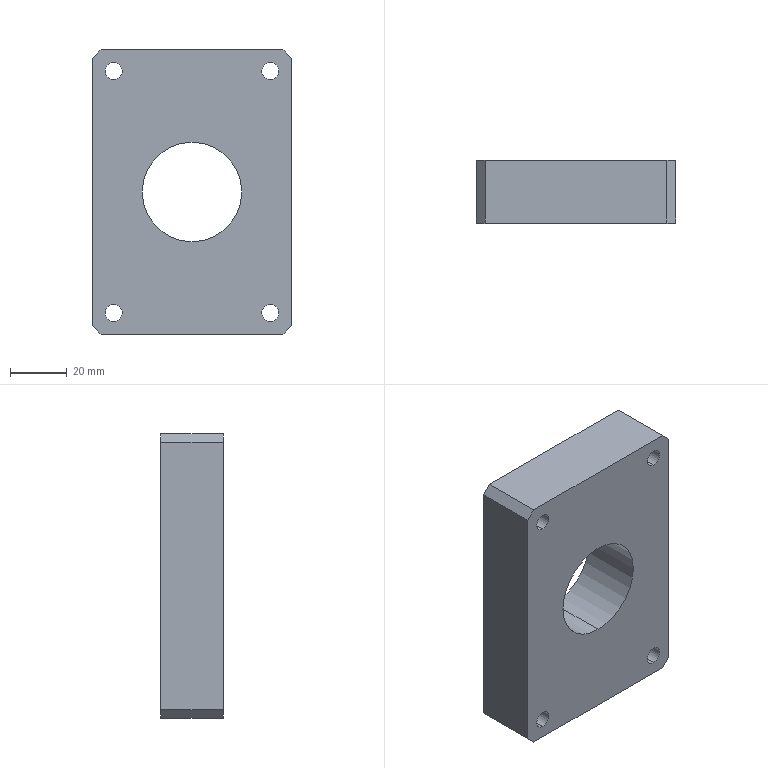Component | SolidWorks | CounterMountingPlate-1 | 1 solid | 35 faces | box 70 x 22 x 100 mm | volume 128818 mm3 | cylinder 20 | plane 15 | commonest cylinder face diameters 6 x10 9 x8 35 x2
build123d program:
from build123d import *

# Parameters (mm, degrees)
SKETCH1_W                                           = 70
SKETCH1_H                                           = 100
BOSS_EXTRUDE1_DEPTH                                 = 22
SKETCH2_R                                           = 17.5
CUT_EXTRUDE1_DEPTH                                  = 65.877
CYLINDRICAL_COUNTERSUNK_HOLE_FOR_M5_HEX_D           = 6
CYLINDRICAL_COUNTERSUNK_HOLE_FOR_M5_HEX_CBORE_D     = 9
CYLINDRICAL_COUNTERSUNK_HOLE_FOR_M5_HEX_CBORE_DEPTH = 6
CHAMFER1_SIZE                                       = 3
SKETCH8_R                                           = 3
CUT_EXTRUDE2_DEPTH                                  = 10


with BuildPart() as part:
    # Sketch1 → Boss-Extrude1 (new body)
    with BuildSketch(Plane(origin=(0, 0, 0), x_dir=(1, 0, 0), z_dir=(0, 1, 0))):
        Rectangle(SKETCH1_W, SKETCH1_H)
    extrude(amount=BOSS_EXTRUDE1_DEPTH)

    # Sketch2 → Cut-Extrude1 (cut, through all)
    with BuildSketch(Plane.XZ):
        with Locations(Location((0, 0, 0), (0, 0, 270))):
            Circle(SKETCH2_R)
    extrude(amount=-CUT_EXTRUDE1_DEPTH, mode=Mode.SUBTRACT)

    # Cylindrical Countersunk Hole for M5 Hex (through all)
    with Locations(Plane(origin=(0, 22, 0), x_dir=(1, 0, 0), z_dir=(0, 1, 0))):
        with Locations((-27.5, 42.5), (27.5, 42.5), (27.5, -42.5), (-27.5, -42.5)):
            CounterBoreHole(CYLINDRICAL_COUNTERSUNK_HOLE_FOR_M5_HEX_D / 2, CYLINDRICAL_COUNTERSUNK_HOLE_FOR_M5_HEX_CBORE_D / 2, CYLINDRICAL_COUNTERSUNK_HOLE_FOR_M5_HEX_CBORE_DEPTH)

    # Chamfer1
    chamfer1_edges = [part.edges().sort_by_distance(p)[0] for p in [
        (35, 11, 50),
        (-35, 11, 50),
        (-35, 11, -50),
        (35, 11, -50),
    ]]
    chamfer(chamfer1_edges, length=CHAMFER1_SIZE)

    # Sketch8 → Cut-Extrude2 (cut)
    with BuildSketch(Plane(origin=(0, 22, 0), x_dir=(1, 0, 0), z_dir=(0, 1, 0))):
        with Locations(Location((0, -30, 0), (0, 0, 270))):
            Circle(SKETCH8_R)
    extrude(amount=-CUT_EXTRUDE2_DEPTH, mode=Mode.SUBTRACT)


solid = part.part

# Placed as in the assembly
solid = solid.moved(Location((-29.507, 247.589, 458), (0, 0, 0)))
STEP:
#1=COLOUR_RGB('',0.7922,0.8196,0.9333);
#2=FILL_AREA_STYLE_COLOUR('',#1);
#3=FILL_AREA_STYLE('',(#2));
#4=SURFACE_STYLE_FILL_AREA(#3);
#5=SURFACE_SIDE_STYLE('',(#4));
#6=SURFACE_STYLE_USAGE(.BOTH.,#5);
#7=PRESENTATION_STYLE_ASSIGNMENT((#6));
#8=CARTESIAN_POINT('',(-1.162,10.22,19.094));
#9=VERTEX_POINT('',#8);
#10=CARTESIAN_POINT('',(-1.162,10.22,19.331));
#11=VERTEX_POINT('',#10);
#12=CARTESIAN_POINT('',(-1.162,10.22,19.213));
#13=DIRECTION('',(0.,1.,0.));
#14=DIRECTION('',(0.,0.,1.));
#15=AXIS2_PLACEMENT_3D('',#12,#13,#14);
#16=CIRCLE('',#15,0.1181);
#17=EDGE_CURVE('',#9,#11,#16,.T.);
#18=ORIENTED_EDGE('',*,*,#17,.F.);
#19=CARTESIAN_POINT('',(-1.162,10.614,19.094));
#20=VERTEX_POINT('',#19);
#21=CARTESIAN_POINT('',(-1.162,10.22,19.094));
#22=DIRECTION('',(0.,1.,0.));
#23=VECTOR('',#22,39.37);
#24=LINE('',#21,#23);
#25=EDGE_CURVE('',#9,#20,#24,.T.);
#26=ORIENTED_EDGE('',*,*,#25,.T.);
#27=CARTESIAN_POINT('',(-1.162,10.614,19.331));
#28=VERTEX_POINT('',#27);
#29=CARTESIAN_POINT('',(-1.162,10.614,19.213));
#30=DIRECTION('',(0.,1.,0.));
#31=DIRECTION('',(0.,0.,1.));
#32=AXIS2_PLACEMENT_3D('',#29,#30,#31);
#33=CIRCLE('',#32,0.1181);
#34=EDGE_CURVE('',#20,#28,#33,.T.);
#35=ORIENTED_EDGE('',*,*,#34,.T.);
#36=CARTESIAN_POINT('',(-1.162,10.22,19.331));
#37=DIRECTION('',(0.,1.,0.));
#38=VECTOR('',#37,39.37);
#39=LINE('',#36,#38);
#40=EDGE_CURVE('',#11,#28,#39,.T.);
#41=ORIENTED_EDGE('',*,*,#40,.F.);
#42=EDGE_LOOP('',(#18,#26,#35,#41));
#43=FACE_OUTER_BOUND('',#42,.T.);
#44=CARTESIAN_POINT('',(-1.162,10.22,19.213));
#45=DIRECTION('',(0.,1.,0.));
#46=DIRECTION('',(0.,0.,1.));
#47=AXIS2_PLACEMENT_3D('',#44,#45,#46);
#48=CYLINDRICAL_SURFACE('',#47,0.1181);
#49=ADVANCED_FACE('',(#43),#48,.F.);
#50=CARTESIAN_POINT('',(-2.244,10.378,16.181));
#51=VERTEX_POINT('',#50);
#52=CARTESIAN_POINT('',(-2.244,10.378,16.535));
#53=VERTEX_POINT('',#52);
#54=CARTESIAN_POINT('',(-2.244,10.378,16.358));
#55=DIRECTION('',(0.,1.,0.));
#56=DIRECTION('',(0.,0.,1.));
#57=AXIS2_PLACEMENT_3D('',#54,#55,#56);
#58=CIRCLE('',#57,0.1772);
#59=EDGE_CURVE('',#51,#53,#58,.T.);
#60=ORIENTED_EDGE('',*,*,#59,.F.);
#61=CARTESIAN_POINT('',(-2.244,10.614,16.181));
#62=VERTEX_POINT('',#61);
#63=CARTESIAN_POINT('',(-2.244,10.614,16.181));
#64=DIRECTION('',(0.,1.,0.));
#65=VECTOR('',#64,39.37);
#66=LINE('',#63,#65);
#67=EDGE_CURVE('',#51,#62,#66,.T.);
#68=ORIENTED_EDGE('',*,*,#67,.T.);
#69=CARTESIAN_POINT('',(-2.244,10.614,16.535));
#70=VERTEX_POINT('',#69);
#71=CARTESIAN_POINT('',(-2.244,10.614,16.358));
#72=DIRECTION('',(0.,1.,0.));
#73=DIRECTION('',(0.,0.,1.));
#74=AXIS2_PLACEMENT_3D('',#71,#72,#73);
#75=CIRCLE('',#74,0.1772);
#76=EDGE_CURVE('',#62,#70,#75,.T.);
#77=ORIENTED_EDGE('',*,*,#76,.T.);
#78=CARTESIAN_POINT('',(-2.244,10.614,16.535));
#79=DIRECTION('',(0.,1.,0.));
#80=VECTOR('',#79,39.37);
#81=LINE('',#78,#80);
#82=EDGE_CURVE('',#53,#70,#81,.T.);
#83=ORIENTED_EDGE('',*,*,#82,.F.);
#84=EDGE_LOOP('',(#60,#68,#77,#83));
#85=FACE_OUTER_BOUND('',#84,.T.);
#86=CARTESIAN_POINT('',(-2.244,10.614,16.358));
#87=DIRECTION('',(0.,1.,0.));
#88=DIRECTION('',(0.,0.,1.));
#89=AXIS2_PLACEMENT_3D('',#86,#87,#88);
#90=CYLINDRICAL_SURFACE('',#89,0.1772);
#91=ADVANCED_FACE('',(#85),#90,.F.);
#92=CARTESIAN_POINT('',(-2.244,9.748,16.24));
#93=VERTEX_POINT('',#92);
#94=CARTESIAN_POINT('',(-2.244,9.748,16.476));
#95=VERTEX_POINT('',#94);
#96=CARTESIAN_POINT('',(-2.244,9.748,16.358));
#97=DIRECTION('',(0.,1.,0.));
#98=DIRECTION('',(0.,0.,1.));
#99=AXIS2_PLACEMENT_3D('',#96,#97,#98);
#100=CIRCLE('',#99,0.1181);
#101=EDGE_CURVE('',#93,#95,#100,.T.);
#102=ORIENTED_EDGE('',*,*,#101,.F.);
#103=CARTESIAN_POINT('',(-2.244,10.378,16.24));
#104=VERTEX_POINT('',#103);
#105=CARTESIAN_POINT('',(-2.244,10.614,16.24));
#106=DIRECTION('',(0.,1.,0.));
#107=VECTOR('',#106,39.37);
#108=LINE('',#105,#107);
#109=EDGE_CURVE('',#93,#104,#108,.T.);
#110=ORIENTED_EDGE('',*,*,#109,.T.);
#111=CARTESIAN_POINT('',(-2.244,10.378,16.476));
#112=VERTEX_POINT('',#111);
#113=CARTESIAN_POINT('',(-2.244,10.378,16.358));
#114=DIRECTION('',(0.,1.,0.));
#115=DIRECTION('',(0.,0.,1.));
#116=AXIS2_PLACEMENT_3D('',#113,#114,#115);
#117=CIRCLE('',#116,0.1181);
#118=EDGE_CURVE('',#104,#112,#117,.T.);
#119=ORIENTED_EDGE('',*,*,#118,.T.);
#120=CARTESIAN_POINT('',(-2.244,10.614,16.476));
#121=DIRECTION('',(0.,1.,0.));
#122=VECTOR('',#121,39.37);
#123=LINE('',#120,#122);
#124=EDGE_CURVE('',#95,#112,#123,.T.);
#125=ORIENTED_EDGE('',*,*,#124,.F.);
#126=EDGE_LOOP('',(#102,#110,#119,#125));
#127=FACE_OUTER_BOUND('',#126,.T.);
#128=CARTESIAN_POINT('',(-2.244,10.614,16.358));
#129=DIRECTION('',(0.,1.,0.));
#130=DIRECTION('',(0.,0.,1.));
#131=AXIS2_PLACEMENT_3D('',#128,#129,#130);
#132=CYLINDRICAL_SURFACE('',#131,0.1181);
#133=ADVANCED_FACE('',(#127),#132,.F.);
#134=CARTESIAN_POINT('',(-0.079,10.378,16.181));
#135=VERTEX_POINT('',#134);
#136=CARTESIAN_POINT('',(-0.079,10.378,16.535));
#137=VERTEX_POINT('',#136);
#138=CARTESIAN_POINT('',(-0.079,10.378,16.358));
#139=DIRECTION('',(0.,1.,0.));
#140=DIRECTION('',(0.,0.,1.));
#141=AXIS2_PLACEMENT_3D('',#138,#139,#140);
#142=CIRCLE('',#141,0.1772);
#143=EDGE_CURVE('',#135,#137,#142,.T.);
#144=ORIENTED_EDGE('',*,*,#143,.F.);
#145=CARTESIAN_POINT('',(-0.079,10.614,16.181));
#146=VERTEX_POINT('',#145);
#147=CARTESIAN_POINT('',(-0.079,10.614,16.181));
#148=DIRECTION('',(0.,1.,0.));
#149=VECTOR('',#148,39.37);
#150=LINE('',#147,#149);
#151=EDGE_CURVE('',#135,#146,#150,.T.);
#152=ORIENTED_EDGE('',*,*,#151,.T.);
#153=CARTESIAN_POINT('',(-0.079,10.614,16.535));
#154=VERTEX_POINT('',#153);
#155=CARTESIAN_POINT('',(-0.079,10.614,16.358));
#156=DIRECTION('',(0.,1.,0.));
#157=DIRECTION('',(0.,0.,1.));
#158=AXIS2_PLACEMENT_3D('',#155,#156,#157);
#159=CIRCLE('',#158,0.1772);
#160=EDGE_CURVE('',#146,#154,#159,.T.);
#161=ORIENTED_EDGE('',*,*,#160,.T.);
#162=CARTESIAN_POINT('',(-0.079,10.614,16.535));
#163=DIRECTION('',(0.,1.,0.));
#164=VECTOR('',#163,39.37);
#165=LINE('',#162,#164);
#166=EDGE_CURVE('',#137,#154,#165,.T.);
#167=ORIENTED_EDGE('',*,*,#166,.F.);
#168=EDGE_LOOP('',(#144,#152,#161,#167));
#169=FACE_OUTER_BOUND('',#168,.T.);
#170=CARTESIAN_POINT('',(-0.079,10.614,16.358));
#171=DIRECTION('',(0.,1.,0.));
#172=DIRECTION('',(0.,0.,1.));
#173=AXIS2_PLACEMENT_3D('',#170,#171,#172);
#174=CYLINDRICAL_SURFACE('',#173,0.1772);
#175=ADVANCED_FACE('',(#169),#174,.F.);
#176=CARTESIAN_POINT('',(-0.079,9.748,16.24));
#177=VERTEX_POINT('',#176);
#178=CARTESIAN_POINT('',(-0.079,9.748,16.476));
#179=VERTEX_POINT('',#178);
#180=CARTESIAN_POINT('',(-0.079,9.748,16.358));
#181=DIRECTION('',(0.,1.,0.));
#182=DIRECTION('',(0.,0.,1.));
#183=AXIS2_PLACEMENT_3D('',#180,#181,#182);
#184=CIRCLE('',#183,0.1181);
#185=EDGE_CURVE('',#177,#179,#184,.T.);
#186=ORIENTED_EDGE('',*,*,#185,.F.);
#187=CARTESIAN_POINT('',(-0.079,10.378,16.24));
#188=VERTEX_POINT('',#187);
#189=CARTESIAN_POINT('',(-0.079,10.614,16.24));
#190=DIRECTION('',(0.,1.,0.));
#191=VECTOR('',#190,39.37);
#192=LINE('',#189,#191);
#193=EDGE_CURVE('',#177,#188,#192,.T.);
#194=ORIENTED_EDGE('',*,*,#193,.T.);
#195=CARTESIAN_POINT('',(-0.079,10.378,16.476));
#196=VERTEX_POINT('',#195);
#197=CARTESIAN_POINT('',(-0.079,10.378,16.358));
#198=DIRECTION('',(0.,1.,0.));
#199=DIRECTION('',(0.,0.,1.));
#200=AXIS2_PLACEMENT_3D('',#197,#198,#199);
#201=CIRCLE('',#200,0.1181);
#202=EDGE_CURVE('',#188,#196,#201,.T.);
#203=ORIENTED_EDGE('',*,*,#202,.T.);
#204=CARTESIAN_POINT('',(-0.079,10.614,16.476));
#205=DIRECTION('',(0.,1.,0.));
#206=VECTOR('',#205,39.37);
#207=LINE('',#204,#206);
#208=EDGE_CURVE('',#179,#196,#207,.T.);
#209=ORIENTED_EDGE('',*,*,#208,.F.);
#210=EDGE_LOOP('',(#186,#194,#203,#209));
#211=FACE_OUTER_BOUND('',#210,.T.);
#212=CARTESIAN_POINT('',(-0.079,10.614,16.358));
#213=DIRECTION('',(0.,1.,0.));
#214=DIRECTION('',(0.,0.,1.));
#215=AXIS2_PLACEMENT_3D('',#212,#213,#214);
#216=CYLINDRICAL_SURFACE('',#215,0.1181);
#217=ADVANCED_FACE('',(#211),#216,.F.);
#218=CARTESIAN_POINT('',(-0.079,10.378,19.528));
#219=VERTEX_POINT('',#218);
#220=CARTESIAN_POINT('',(-0.079,10.378,19.882));
#221=VERTEX_POINT('',#220);
#222=CARTESIAN_POINT('',(-0.079,10.378,19.705));
#223=DIRECTION('',(0.,1.,0.));
#224=DIRECTION('',(0.,0.,1.));
#225=AXIS2_PLACEMENT_3D('',#222,#223,#224);
#226=CIRCLE('',#225,0.1772);
#227=EDGE_CURVE('',#219,#221,#226,.T.);
#228=ORIENTED_EDGE('',*,*,#227,.F.);
#229=CARTESIAN_POINT('',(-0.079,10.614,19.528));
#230=VERTEX_POINT('',#229);
#231=CARTESIAN_POINT('',(-0.079,10.614,19.528));
#232=DIRECTION('',(0.,1.,0.));
#233=VECTOR('',#232,39.37);
#234=LINE('',#231,#233);
#235=EDGE_CURVE('',#219,#230,#234,.T.);
#236=ORIENTED_EDGE('',*,*,#235,.T.);
#237=CARTESIAN_POINT('',(-0.079,10.614,19.882));
#238=VERTEX_POINT('',#237);
#239=CARTESIAN_POINT('',(-0.079,10.614,19.705));
#240=DIRECTION('',(0.,1.,0.));
#241=DIRECTION('',(0.,0.,1.));
#242=AXIS2_PLACEMENT_3D('',#239,#240,#241);
#243=CIRCLE('',#242,0.1772);
#244=EDGE_CURVE('',#230,#238,#243,.T.);
#245=ORIENTED_EDGE('',*,*,#244,.T.);
#246=CARTESIAN_POINT('',(-0.079,10.614,19.882));
#247=DIRECTION('',(0.,1.,0.));
#248=VECTOR('',#247,39.37);
#249=LINE('',#246,#248);
#250=EDGE_CURVE('',#221,#238,#249,.T.);
#251=ORIENTED_EDGE('',*,*,#250,.F.);
#252=EDGE_LOOP('',(#228,#236,#245,#251));
#253=FACE_OUTER_BOUND('',#252,.T.);
#254=CARTESIAN_POINT('',(-0.079,10.614,19.705));
#255=DIRECTION('',(0.,1.,0.));
#256=DIRECTION('',(0.,0.,1.));
#257=AXIS2_PLACEMENT_3D('',#254,#255,#256);
#258=CYLINDRICAL_SURFACE('',#257,0.1772);
#259=ADVANCED_FACE('',(#253),#258,.F.);
#260=CARTESIAN_POINT('',(-0.079,9.748,19.587));
#261=VERTEX_POINT('',#260);
#262=CARTESIAN_POINT('',(-0.079,9.748,19.823));
#263=VERTEX_POINT('',#262);
#264=CARTESIAN_POINT('',(-0.079,9.748,19.705));
#265=DIRECTION('',(0.,1.,0.));
#266=DIRECTION('',(0.,0.,1.));
#267=AXIS2_PLACEMENT_3D('',#264,#265,#266);
#268=CIRCLE('',#267,0.1181);
#269=EDGE_CURVE('',#261,#263,#268,.T.);
#270=ORIENTED_EDGE('',*,*,#269,.F.);
#271=CARTESIAN_POINT('',(-0.079,10.378,19.587));
#272=VERTEX_POINT('',#271);
#273=CARTESIAN_POINT('',(-0.079,10.614,19.587));
#274=DIRECTION('',(0.,1.,0.));
#275=VECTOR('',#274,39.37);
#276=LINE('',#273,#275);
#277=EDGE_CURVE('',#261,#272,#276,.T.);
#278=ORIENTED_EDGE('',*,*,#277,.T.);
#279=CARTESIAN_POINT('',(-0.079,10.378,19.823));
#280=VERTEX_POINT('',#279);
#281=CARTESIAN_POINT('',(-0.079,10.378,19.705));
#282=DIRECTION('',(0.,1.,0.));
#283=DIRECTION('',(0.,0.,1.));
#284=AXIS2_PLACEMENT_3D('',#281,#282,#283);
#285=CIRCLE('',#284,0.1181);
#286=EDGE_CURVE('',#272,#280,#285,.T.);
#287=ORIENTED_EDGE('',*,*,#286,.T.);
#288=CARTESIAN_POINT('',(-0.079,10.614,19.823));
#289=DIRECTION('',(0.,1.,0.));
#290=VECTOR('',#289,39.37);
#291=LINE('',#288,#290);
#292=EDGE_CURVE('',#263,#280,#291,.T.);
#293=ORIENTED_EDGE('',*,*,#292,.F.);
#294=EDGE_LOOP('',(#270,#278,#287,#293));
#295=FACE_OUTER_BOUND('',#294,.T.);
#296=CARTESIAN_POINT('',(-0.079,10.614,19.705));
#297=DIRECTION('',(0.,1.,0.));
#298=DIRECTION('',(0.,0.,1.));
#299=AXIS2_PLACEMENT_3D('',#296,#297,#298);
#300=CYLINDRICAL_SURFACE('',#299,0.1181);
#301=ADVANCED_FACE('',(#295),#300,.F.);
#302=CARTESIAN_POINT('',(-2.244,10.378,19.528));
#303=VERTEX_POINT('',#302);
#304=CARTESIAN_POINT('',(-2.244,10.378,19.882));
#305=VERTEX_POINT('',#304);
#306=CARTESIAN_POINT('',(-2.244,10.378,19.705));
#307=DIRECTION('',(0.,1.,0.));
#308=DIRECTION('',(0.,0.,1.));
#309=AXIS2_PLACEMENT_3D('',#306,#307,#308);
#310=CIRCLE('',#309,0.1772);
#311=EDGE_CURVE('',#303,#305,#310,.T.);
#312=ORIENTED_EDGE('',*,*,#311,.F.);
#313=CARTESIAN_POINT('',(-2.244,10.614,19.528));
#314=VERTEX_POINT('',#313);
#315=CARTESIAN_POINT('',(-2.244,10.614,19.528));
#316=DIRECTION('',(0.,1.,0.));
#317=VECTOR('',#316,39.37);
#318=LINE('',#315,#317);
#319=EDGE_CURVE('',#303,#314,#318,.T.);
#320=ORIENTED_EDGE('',*,*,#319,.T.);
#321=CARTESIAN_POINT('',(-2.244,10.614,19.882));
#322=VERTEX_POINT('',#321);
#323=CARTESIAN_POINT('',(-2.244,10.614,19.705));
#324=DIRECTION('',(0.,1.,0.));
#325=DIRECTION('',(0.,0.,1.));
#326=AXIS2_PLACEMENT_3D('',#323,#324,#325);
#327=CIRCLE('',#326,0.1772);
#328=EDGE_CURVE('',#314,#322,#327,.T.);
#329=ORIENTED_EDGE('',*,*,#328,.T.);
#330=CARTESIAN_POINT('',(-2.244,10.614,19.882));
#331=DIRECTION('',(0.,1.,0.));
#332=VECTOR('',#331,39.37);
#333=LINE('',#330,#332);
#334=EDGE_CURVE('',#305,#322,#333,.T.);
#335=ORIENTED_EDGE('',*,*,#334,.F.);
#336=EDGE_LOOP('',(#312,#320,#329,#335));
#337=FACE_OUTER_BOUND('',#336,.T.);
#338=CARTESIAN_POINT('',(-2.244,10.614,19.705));
#339=DIRECTION('',(0.,1.,0.));
#340=DIRECTION('',(0.,0.,1.));
#341=AXIS2_PLACEMENT_3D('',#338,#339,#340);
#342=CYLINDRICAL_SURFACE('',#341,0.1772);
#343=ADVANCED_FACE('',(#337),#342,.F.);
#344=CARTESIAN_POINT('',(-2.244,9.748,19.587));
#345=VERTEX_POINT('',#344);
#346=CARTESIAN_POINT('',(-2.244,9.748,19.823));
#347=VERTEX_POINT('',#346);
#348=CARTESIAN_POINT('',(-2.244,9.748,19.705));
#349=DIRECTION('',(0.,1.,0.));
#350=DIRECTION('',(0.,0.,1.));
#351=AXIS2_PLACEMENT_3D('',#348,#349,#350);
#352=CIRCLE('',#351,0.1181);
#353=EDGE_CURVE('',#345,#347,#352,.T.);
#354=ORIENTED_EDGE('',*,*,#353,.F.);
#355=CARTESIAN_POINT('',(-2.244,10.378,19.587));
#356=VERTEX_POINT('',#355);
#357=CARTESIAN_POINT('',(-2.244,10.614,19.587));
#358=DIRECTION('',(0.,1.,0.));
#359=VECTOR('',#358,39.37);
#360=LINE('',#357,#359);
#361=EDGE_CURVE('',#345,#356,#360,.T.);
#362=ORIENTED_EDGE('',*,*,#361,.T.);
#363=CARTESIAN_POINT('',(-2.244,10.378,19.823));
#364=VERTEX_POINT('',#363);
#365=CARTESIAN_POINT('',(-2.244,10.378,19.705));
#366=DIRECTION('',(0.,1.,0.));
#367=DIRECTION('',(0.,0.,1.));
#368=AXIS2_PLACEMENT_3D('',#365,#366,#367);
#369=CIRCLE('',#368,0.1181);
#370=EDGE_CURVE('',#356,#364,#369,.T.);
#371=ORIENTED_EDGE('',*,*,#370,.T.);
#372=CARTESIAN_POINT('',(-2.244,10.614,19.823));
#373=DIRECTION('',(0.,1.,0.));
#374=VECTOR('',#373,39.37);
#375=LINE('',#372,#374);
#376=EDGE_CURVE('',#347,#364,#375,.T.);
#377=ORIENTED_EDGE('',*,*,#376,.F.);
#378=EDGE_LOOP('',(#354,#362,#371,#377));
#379=FACE_OUTER_BOUND('',#378,.T.);
#380=CARTESIAN_POINT('',(-2.244,10.614,19.705));
#381=DIRECTION('',(0.,1.,0.));
#382=DIRECTION('',(0.,0.,1.));
#383=AXIS2_PLACEMENT_3D('',#380,#381,#382);
#384=CYLINDRICAL_SURFACE('',#383,0.1181);
#385=ADVANCED_FACE('',(#379),#384,.F.);
#386=CARTESIAN_POINT('',(-1.162,10.614,18.72));
#387=VERTEX_POINT('',#386);
#388=CARTESIAN_POINT('',(-1.162,10.614,17.343));
#389=VERTEX_POINT('',#388);
#390=CARTESIAN_POINT('',(-1.162,10.614,18.031));
#391=DIRECTION('',(0.,-1.,0.));
#392=DIRECTION('',(0.,0.,-1.));
#393=AXIS2_PLACEMENT_3D('',#390,#391,#392);
#394=CIRCLE('',#393,0.689);
#395=EDGE_CURVE('',#387,#389,#394,.T.);
#396=ORIENTED_EDGE('',*,*,#395,.F.);
#397=CARTESIAN_POINT('',(-1.162,9.748,18.72));
#398=VERTEX_POINT('',#397);
#399=CARTESIAN_POINT('',(-1.162,10.614,18.72));
#400=DIRECTION('',(0.,-1.,0.));
#401=VECTOR('',#400,39.37);
#402=LINE('',#399,#401);
#403=EDGE_CURVE('',#387,#398,#402,.T.);
#404=ORIENTED_EDGE('',*,*,#403,.T.);
#405=CARTESIAN_POINT('',(-1.162,9.748,17.343));
#406=VERTEX_POINT('',#405);
#407=CARTESIAN_POINT('',(-1.162,9.748,18.031));
#408=DIRECTION('',(0.,-1.,0.));
#409=DIRECTION('',(0.,0.,-1.));
#410=AXIS2_PLACEMENT_3D('',#407,#408,#409);
#411=CIRCLE('',#410,0.689);
#412=EDGE_CURVE('',#398,#406,#411,.T.);
#413=ORIENTED_EDGE('',*,*,#412,.T.);
#414=CARTESIAN_POINT('',(-1.162,10.614,17.343));
#415=DIRECTION('',(0.,-1.,0.));
#416=VECTOR('',#415,39.37);
#417=LINE('',#414,#416);
#418=EDGE_CURVE('',#389,#406,#417,.T.);
#419=ORIENTED_EDGE('',*,*,#418,.F.);
#420=EDGE_LOOP('',(#396,#404,#413,#419));
#421=FACE_OUTER_BOUND('',#420,.T.);
#422=CARTESIAN_POINT('',(-1.162,10.614,18.031));
#423=DIRECTION('',(0.,-1.,0.));
#424=DIRECTION('',(0.,0.,-1.));
#425=AXIS2_PLACEMENT_3D('',#422,#423,#424);
#426=CYLINDRICAL_SURFACE('',#425,0.689);
#427=ADVANCED_FACE('',(#421),#426,.F.);
#428=CARTESIAN_POINT('',(0.2163,9.748,19.882));
#429=VERTEX_POINT('',#428);
#430=CARTESIAN_POINT('',(0.2163,9.748,16.181));
#431=VERTEX_POINT('',#430);
#432=CARTESIAN_POINT('',(0.2163,9.748,16.063));
#433=DIRECTION('',(-0.,0.,-1.));
#434=VECTOR('',#433,39.37);
#435=LINE('',#432,#434);
#436=EDGE_CURVE('',#429,#431,#435,.T.);
#437=ORIENTED_EDGE('',*,*,#436,.T.);
#438=CARTESIAN_POINT('',(0.2163,10.614,16.181));
#439=VERTEX_POINT('',#438);
#440=CARTESIAN_POINT('',(0.2163,10.614,16.181));
#441=DIRECTION('',(0.,1.,0.));
#442=VECTOR('',#441,39.37);
#443=LINE('',#440,#442);
#444=EDGE_CURVE('',#431,#439,#443,.T.);
#445=ORIENTED_EDGE('',*,*,#444,.T.);
#446=CARTESIAN_POINT('',(0.2163,10.614,19.882));
#447=VERTEX_POINT('',#446);
#448=CARTESIAN_POINT('',(0.2163,10.614,16.063));
#449=DIRECTION('',(-0.,0.,-1.));
#450=VECTOR('',#449,39.37);
#451=LINE('',#448,#450);
#452=EDGE_CURVE('',#447,#439,#451,.T.);
#453=ORIENTED_EDGE('',*,*,#452,.F.);
#454=CARTESIAN_POINT('',(0.2163,10.614,19.882));
#455=DIRECTION('',(0.,-1.,0.));
#456=VECTOR('',#455,39.37);
#457=LINE('',#454,#456);
#458=EDGE_CURVE('',#447,#429,#457,.T.);
#459=ORIENTED_EDGE('',*,*,#458,.T.);
#460=EDGE_LOOP('',(#437,#445,#453,#459));
#461=FACE_OUTER_BOUND('',#460,.T.);
#462=CARTESIAN_POINT('',(0.2163,10.614,16.063));
#463=DIRECTION('',(-1.,0.,0.));
#464=DIRECTION('',(0.,0.,1.));
#465=AXIS2_PLACEMENT_3D('',#462,#463,#464);
#466=PLANE('',#465);
#467=ADVANCED_FACE('',(#461),#466,.F.);
#468=CARTESIAN_POINT('',(0.09817,9.748,16.063));
#469=VERTEX_POINT('',#468);
#470=CARTESIAN_POINT('',(-2.422,9.748,16.063));
#471=VERTEX_POINT('',#470);
#472=CARTESIAN_POINT('',(-2.54,9.748,16.063));
#473=DIRECTION('',(-1.,0.,0.));
#474=VECTOR('',#473,39.37);
#475=LINE('',#472,#474);
#476=EDGE_CURVE('',#469,#471,#475,.T.);
#477=ORIENTED_EDGE('',*,*,#476,.T.);
#478=CARTESIAN_POINT('',(-2.422,10.614,16.063));
#479=VERTEX_POINT('',#478);
#480=CARTESIAN_POINT('',(-2.422,10.614,16.063));
#481=DIRECTION('',(0.,1.,0.));
#482=VECTOR('',#481,39.37);
#483=LINE('',#480,#482);
#484=EDGE_CURVE('',#471,#479,#483,.T.);
#485=ORIENTED_EDGE('',*,*,#484,.T.);
#486=CARTESIAN_POINT('',(0.09817,10.614,16.063));
#487=VERTEX_POINT('',#486);
#488=CARTESIAN_POINT('',(-2.54,10.614,16.063));
#489=DIRECTION('',(-1.,0.,0.));
#490=VECTOR('',#489,39.37);
#491=LINE('',#488,#490);
#492=EDGE_CURVE('',#487,#479,#491,.T.);
#493=ORIENTED_EDGE('',*,*,#492,.F.);
#494=CARTESIAN_POINT('',(0.09817,10.614,16.063));
#495=DIRECTION('',(0.,-1.,0.));
#496=VECTOR('',#495,39.37);
#497=LINE('',#494,#496);
#498=EDGE_CURVE('',#487,#469,#497,.T.);
#499=ORIENTED_EDGE('',*,*,#498,.T.);
#500=EDGE_LOOP('',(#477,#485,#493,#499));
#501=FACE_OUTER_BOUND('',#500,.T.);
#502=CARTESIAN_POINT('',(-2.54,10.614,16.063));
#503=DIRECTION('',(0.,0.,1.));
#504=DIRECTION('',(1.,0.,0.));
#505=AXIS2_PLACEMENT_3D('',#502,#503,#504);
#506=PLANE('',#505);
#507=ADVANCED_FACE('',(#501),#506,.F.);
#508=CARTESIAN_POINT('',(-2.54,10.614,16.181));
#509=VERTEX_POINT('',#508);
#510=CARTESIAN_POINT('',(-2.54,10.614,19.882));
#511=VERTEX_POINT('',#510);
#512=CARTESIAN_POINT('',(-2.54,10.614,16.063));
#513=DIRECTION('',(0.,0.,1.));
#514=VECTOR('',#513,39.37);
#515=LINE('',#512,#514);
#516=EDGE_CURVE('',#509,#511,#515,.T.);
#517=ORIENTED_EDGE('',*,*,#516,.F.);
#518=CARTESIAN_POINT('',(-2.54,9.748,16.181));
#519=VERTEX_POINT('',#518);
#520=CARTESIAN_POINT('',(-2.54,10.614,16.181));
#521=DIRECTION('',(0.,-1.,0.));
#522=VECTOR('',#521,39.37);
#523=LINE('',#520,#522);
#524=EDGE_CURVE('',#509,#519,#523,.T.);
#525=ORIENTED_EDGE('',*,*,#524,.T.);
#526=CARTESIAN_POINT('',(-2.54,9.748,19.882));
#527=VERTEX_POINT('',#526);
#528=CARTESIAN_POINT('',(-2.54,9.748,16.063));
#529=DIRECTION('',(0.,0.,1.));
#530=VECTOR('',#529,39.37);
#531=LINE('',#528,#530);
#532=EDGE_CURVE('',#519,#527,#531,.T.);
#533=ORIENTED_EDGE('',*,*,#532,.T.);
#534=CARTESIAN_POINT('',(-2.54,10.614,19.882));
#535=DIRECTION('',(0.,1.,0.));
#536=VECTOR('',#535,39.37);
#537=LINE('',#534,#536);
#538=EDGE_CURVE('',#527,#511,#537,.T.);
#539=ORIENTED_EDGE('',*,*,#538,.T.);
#540=EDGE_LOOP('',(#517,#525,#533,#539));
#541=FACE_OUTER_BOUND('',#540,.T.);
#542=CARTESIAN_POINT('',(-2.54,10.614,16.063));
#543=DIRECTION('',(1.,0.,-0.));
#544=DIRECTION('',(-0.,0.,-1.));
#545=AXIS2_PLACEMENT_3D('',#542,#543,#544);
#546=PLANE('',#545);
#547=ADVANCED_FACE('',(#541),#546,.F.);
#548=CARTESIAN_POINT('',(-2.422,10.614,20.));
#549=VERTEX_POINT('',#548);
#550=CARTESIAN_POINT('',(0.09817,10.614,20.));
#551=VERTEX_POINT('',#550);
#552=CARTESIAN_POINT('',(-2.54,10.614,20.));
#553=DIRECTION('',(1.,0.,0.));
#554=VECTOR('',#553,39.37);
#555=LINE('',#552,#554);
#556=EDGE_CURVE('',#549,#551,#555,.T.);
#557=ORIENTED_EDGE('',*,*,#556,.F.);
#558=CARTESIAN_POINT('',(-2.422,9.748,20.));
#559=VERTEX_POINT('',#558);
#560=CARTESIAN_POINT('',(-2.422,10.614,20.));
#561=DIRECTION('',(0.,-1.,0.));
#562=VECTOR('',#561,39.37);
#563=LINE('',#560,#562);
#564=EDGE_CURVE('',#549,#559,#563,.T.);
#565=ORIENTED_EDGE('',*,*,#564,.T.);
#566=CARTESIAN_POINT('',(0.09817,9.748,20.));
#567=VERTEX_POINT('',#566);
#568=CARTESIAN_POINT('',(-2.54,9.748,20.));
#569=DIRECTION('',(1.,0.,0.));
#570=VECTOR('',#569,39.37);
#571=LINE('',#568,#570);
#572=EDGE_CURVE('',#559,#567,#571,.T.);
#573=ORIENTED_EDGE('',*,*,#572,.T.);
#574=CARTESIAN_POINT('',(0.09817,10.614,20.));
#575=DIRECTION('',(0.,1.,0.));
#576=VECTOR('',#575,39.37);
#577=LINE('',#574,#576);
#578=EDGE_CURVE('',#567,#551,#577,.T.);
#579=ORIENTED_EDGE('',*,*,#578,.T.);
#580=EDGE_LOOP('',(#557,#565,#573,#579));
#581=FACE_OUTER_BOUND('',#580,.T.);
#582=CARTESIAN_POINT('',(-2.54,10.614,20.));
#583=DIRECTION('',(0.,0.,-1.));
#584=DIRECTION('',(-1.,0.,0.));
#585=AXIS2_PLACEMENT_3D('',#582,#583,#584);
#586=PLANE('',#585);
#587=ADVANCED_FACE('',(#581),#586,.F.);
#588=CARTESIAN_POINT('',(-1.162,10.614,19.213));
#589=DIRECTION('',(0.,1.,0.));
#590=DIRECTION('',(0.,0.,1.));
#591=AXIS2_PLACEMENT_3D('',#588,#589,#590);
#592=CIRCLE('',#591,0.1181);
#593=EDGE_CURVE('',#28,#20,#592,.T.);
#594=ORIENTED_EDGE('',*,*,#593,.F.);
#595=ORIENTED_EDGE('',*,*,#34,.F.);
#596=EDGE_LOOP('',(#594,#595));
#597=FACE_BOUND('',#596,.T.);
#598=CARTESIAN_POINT('',(-2.244,10.614,16.358));
#599=DIRECTION('',(0.,1.,0.));
#600=DIRECTION('',(0.,0.,1.));
#601=AXIS2_PLACEMENT_3D('',#598,#599,#600);
#602=CIRCLE('',#601,0.1772);
#603=EDGE_CURVE('',#70,#62,#602,.T.);
#604=ORIENTED_EDGE('',*,*,#603,.F.);
#605=ORIENTED_EDGE('',*,*,#76,.F.);
#606=EDGE_LOOP('',(#604,#605));
#607=FACE_BOUND('',#606,.T.);
#608=CARTESIAN_POINT('',(-0.079,10.614,16.358));
#609=DIRECTION('',(0.,1.,0.));
#610=DIRECTION('',(0.,0.,1.));
#611=AXIS2_PLACEMENT_3D('',#608,#609,#610);
#612=CIRCLE('',#611,0.1772);
#613=EDGE_CURVE('',#154,#146,#612,.T.);
#614=ORIENTED_EDGE('',*,*,#613,.F.);
#615=ORIENTED_EDGE('',*,*,#160,.F.);
#616=EDGE_LOOP('',(#614,#615));
#617=FACE_BOUND('',#616,.T.);
#618=CARTESIAN_POINT('',(-0.079,10.614,19.705));
#619=DIRECTION('',(0.,1.,0.));
#620=DIRECTION('',(0.,0.,1.));
#621=AXIS2_PLACEMENT_3D('',#618,#619,#620);
#622=CIRCLE('',#621,0.1772);
#623=EDGE_CURVE('',#238,#230,#622,.T.);
#624=ORIENTED_EDGE('',*,*,#623,.F.);
#625=ORIENTED_EDGE('',*,*,#244,.F.);
#626=EDGE_LOOP('',(#624,#625));
#627=FACE_BOUND('',#626,.T.);
#628=CARTESIAN_POINT('',(-2.244,10.614,19.705));
#629=DIRECTION('',(0.,1.,0.));
#630=DIRECTION('',(0.,0.,1.));
#631=AXIS2_PLACEMENT_3D('',#628,#629,#630);
#632=CIRCLE('',#631,0.1772);
#633=EDGE_CURVE('',#322,#314,#632,.T.);
#634=ORIENTED_EDGE('',*,*,#633,.F.);
#635=ORIENTED_EDGE('',*,*,#328,.F.);
#636=EDGE_LOOP('',(#634,#635));
#637=FACE_BOUND('',#636,.T.);
#638=CARTESIAN_POINT('',(-1.162,10.614,18.031));
#639=DIRECTION('',(0.,-1.,0.));
#640=DIRECTION('',(0.,0.,-1.));
#641=AXIS2_PLACEMENT_3D('',#638,#639,#640);
#642=CIRCLE('',#641,0.689);
#643=EDGE_CURVE('',#389,#387,#642,.T.);
#644=ORIENTED_EDGE('',*,*,#643,.T.);
#645=ORIENTED_EDGE('',*,*,#395,.T.);
#646=EDGE_LOOP('',(#644,#645));
#647=FACE_BOUND('',#646,.T.);
#648=ORIENTED_EDGE('',*,*,#492,.T.);
#649=CARTESIAN_POINT('',(-2.776,10.614,16.417));
#650=DIRECTION('',(-0.7071,0.,0.7071));
#651=VECTOR('',#650,39.37);
#652=LINE('',#649,#651);
#653=EDGE_CURVE('',#479,#509,#652,.T.);
#654=ORIENTED_EDGE('',*,*,#653,.T.);
#655=ORIENTED_EDGE('',*,*,#516,.T.);
#656=CARTESIAN_POINT('',(-2.776,10.614,19.646));
#657=DIRECTION('',(0.7071,0.,0.7071));
#658=VECTOR('',#657,39.37);
#659=LINE('',#656,#658);
#660=EDGE_CURVE('',#511,#549,#659,.T.);
#661=ORIENTED_EDGE('',*,*,#660,.T.);
#662=ORIENTED_EDGE('',*,*,#556,.T.);
#663=CARTESIAN_POINT('',(0.4525,10.614,19.646));
#664=DIRECTION('',(0.7071,0.,-0.7071));
#665=VECTOR('',#664,39.37);
#666=LINE('',#663,#665);
#667=EDGE_CURVE('',#551,#447,#666,.T.);
#668=ORIENTED_EDGE('',*,*,#667,.T.);
#669=ORIENTED_EDGE('',*,*,#452,.T.);
#670=CARTESIAN_POINT('',(0.4525,10.614,16.417));
#671=DIRECTION('',(-0.7071,0.,-0.7071));
#672=VECTOR('',#671,39.37);
#673=LINE('',#670,#672);
#674=EDGE_CURVE('',#439,#487,#673,.T.);
#675=ORIENTED_EDGE('',*,*,#674,.T.);
#676=EDGE_LOOP('',(#648,#654,#655,#661,#662,#668,#669,#675));
#677=FACE_OUTER_BOUND('',#676,.T.);
#678=CARTESIAN_POINT('',(-1.162,10.614,18.031));
#679=DIRECTION('',(0.,1.,0.));
#680=DIRECTION('',(0.,0.,1.));
#681=AXIS2_PLACEMENT_3D('',#678,#679,#680);
#682=PLANE('',#681);
#683=ADVANCED_FACE('',(#597,#607,#617,#627,#637,#647,#677),#682,.T.);
#684=CARTESIAN_POINT('',(-2.244,9.748,16.358));
#685=DIRECTION('',(0.,1.,0.));
#686=DIRECTION('',(0.,0.,1.));
#687=AXIS2_PLACEMENT_3D('',#684,#685,#686);
#688=CIRCLE('',#687,0.1181);
#689=EDGE_CURVE('',#95,#93,#688,.T.);
#690=ORIENTED_EDGE('',*,*,#689,.T.);
#691=ORIENTED_EDGE('',*,*,#101,.T.);
#692=EDGE_LOOP('',(#690,#691));
#693=FACE_BOUND('',#692,.T.);
#694=CARTESIAN_POINT('',(-0.079,9.748,16.358));
#695=DIRECTION('',(0.,1.,0.));
#696=DIRECTION('',(0.,0.,1.));
#697=AXIS2_PLACEMENT_3D('',#694,#695,#696);
#698=CIRCLE('',#697,0.1181);
#699=EDGE_CURVE('',#179,#177,#698,.T.);
#700=ORIENTED_EDGE('',*,*,#699,.T.);
#701=ORIENTED_EDGE('',*,*,#185,.T.);
#702=EDGE_LOOP('',(#700,#701));
#703=FACE_BOUND('',#702,.T.);
#704=CARTESIAN_POINT('',(-0.079,9.748,19.705));
#705=DIRECTION('',(0.,1.,0.));
#706=DIRECTION('',(0.,0.,1.));
#707=AXIS2_PLACEMENT_3D('',#704,#705,#706);
#708=CIRCLE('',#707,0.1181);
#709=EDGE_CURVE('',#263,#261,#708,.T.);
#710=ORIENTED_EDGE('',*,*,#709,.T.);
#711=ORIENTED_EDGE('',*,*,#269,.T.);
#712=EDGE_LOOP('',(#710,#711));
#713=FACE_BOUND('',#712,.T.);
#714=CARTESIAN_POINT('',(-2.244,9.748,19.705));
#715=DIRECTION('',(0.,1.,0.));
#716=DIRECTION('',(0.,0.,1.));
#717=AXIS2_PLACEMENT_3D('',#714,#715,#716);
#718=CIRCLE('',#717,0.1181);
#719=EDGE_CURVE('',#347,#345,#718,.T.);
#720=ORIENTED_EDGE('',*,*,#719,.T.);
#721=ORIENTED_EDGE('',*,*,#353,.T.);
#722=EDGE_LOOP('',(#720,#721));
#723=FACE_BOUND('',#722,.T.);
#724=CARTESIAN_POINT('',(-1.162,9.748,18.031));
#725=DIRECTION('',(0.,-1.,0.));
#726=DIRECTION('',(0.,0.,-1.));
#727=AXIS2_PLACEMENT_3D('',#724,#725,#726);
#728=CIRCLE('',#727,0.689);
#729=EDGE_CURVE('',#406,#398,#728,.T.);
#730=ORIENTED_EDGE('',*,*,#729,.F.);
#731=ORIENTED_EDGE('',*,*,#412,.F.);
#732=EDGE_LOOP('',(#730,#731));
#733=FACE_BOUND('',#732,.T.);
#734=ORIENTED_EDGE('',*,*,#532,.F.);
#735=CARTESIAN_POINT('',(-2.54,9.748,16.181));
#736=DIRECTION('',(0.7071,0.,-0.7071));
#737=VECTOR('',#736,39.37);
#738=LINE('',#735,#737);
#739=EDGE_CURVE('',#519,#471,#738,.T.);
#740=ORIENTED_EDGE('',*,*,#739,.T.);
#741=ORIENTED_EDGE('',*,*,#476,.F.);
#742=CARTESIAN_POINT('',(0.09817,9.748,16.063));
#743=DIRECTION('',(0.7071,0.,0.7071));
#744=VECTOR('',#743,39.37);
#745=LINE('',#742,#744);
#746=EDGE_CURVE('',#469,#431,#745,.T.);
#747=ORIENTED_EDGE('',*,*,#746,.T.);
#748=ORIENTED_EDGE('',*,*,#436,.F.);
#749=CARTESIAN_POINT('',(0.2163,9.748,19.882));
#750=DIRECTION('',(-0.7071,0.,0.7071));
#751=VECTOR('',#750,39.37);
#752=LINE('',#749,#751);
#753=EDGE_CURVE('',#429,#567,#752,.T.);
#754=ORIENTED_EDGE('',*,*,#753,.T.);
#755=ORIENTED_EDGE('',*,*,#572,.F.);
#756=CARTESIAN_POINT('',(-2.422,9.748,20.));
#757=DIRECTION('',(-0.7071,0.,-0.7071));
#758=VECTOR('',#757,39.37);
#759=LINE('',#756,#758);
#760=EDGE_CURVE('',#559,#527,#759,.T.);
#761=ORIENTED_EDGE('',*,*,#760,.T.);
#762=EDGE_LOOP('',(#734,#740,#741,#747,#748,#754,#755,#761));
#763=FACE_OUTER_BOUND('',#762,.T.);
#764=CARTESIAN_POINT('',(-1.162,9.748,18.031));
#765=DIRECTION('',(0.,1.,0.));
#766=DIRECTION('',(0.,0.,1.));
#767=AXIS2_PLACEMENT_3D('',#764,#765,#766);
#768=PLANE('',#767);
#769=ADVANCED_FACE('',(#693,#703,#713,#723,#733,#763),#768,.F.);
#770=ORIENTED_EDGE('',*,*,#403,.F.);
#771=ORIENTED_EDGE('',*,*,#643,.F.);
#772=ORIENTED_EDGE('',*,*,#418,.T.);
#773=ORIENTED_EDGE('',*,*,#729,.T.);
#774=EDGE_LOOP('',(#770,#771,#772,#773));
#775=FACE_OUTER_BOUND('',#774,.T.);
#776=CARTESIAN_POINT('',(-1.162,10.614,18.031));
#777=DIRECTION('',(0.,-1.,0.));
#778=DIRECTION('',(0.,0.,-1.));
#779=AXIS2_PLACEMENT_3D('',#776,#777,#778);
#780=CYLINDRICAL_SURFACE('',#779,0.689);
#781=ADVANCED_FACE('',(#775),#780,.F.);
#782=ORIENTED_EDGE('',*,*,#361,.F.);
#783=ORIENTED_EDGE('',*,*,#719,.F.);
#784=ORIENTED_EDGE('',*,*,#376,.T.);
#785=CARTESIAN_POINT('',(-2.244,10.378,19.705));
#786=DIRECTION('',(0.,1.,0.));
#787=DIRECTION('',(0.,0.,1.));
#788=AXIS2_PLACEMENT_3D('',#785,#786,#787);
#789=CIRCLE('',#788,0.1181);
#790=EDGE_CURVE('',#364,#356,#789,.T.);
#791=ORIENTED_EDGE('',*,*,#790,.T.);
#792=EDGE_LOOP('',(#782,#783,#784,#791));
#793=FACE_OUTER_BOUND('',#792,.T.);
#794=CARTESIAN_POINT('',(-2.244,10.614,19.705));
#795=DIRECTION('',(0.,1.,0.));
#796=DIRECTION('',(0.,0.,1.));
#797=AXIS2_PLACEMENT_3D('',#794,#795,#796);
#798=CYLINDRICAL_SURFACE('',#797,0.1181);
#799=ADVANCED_FACE('',(#793),#798,.F.);
#800=ORIENTED_EDGE('',*,*,#790,.F.);
#801=ORIENTED_EDGE('',*,*,#370,.F.);
#802=EDGE_LOOP('',(#800,#801));
#803=FACE_BOUND('',#802,.T.);
#804=CARTESIAN_POINT('',(-2.244,10.378,19.705));
#805=DIRECTION('',(0.,1.,0.));
#806=DIRECTION('',(0.,0.,1.));
#807=AXIS2_PLACEMENT_3D('',#804,#805,#806);
#808=CIRCLE('',#807,0.1772);
#809=EDGE_CURVE('',#305,#303,#808,.T.);
#810=ORIENTED_EDGE('',*,*,#809,.T.);
#811=ORIENTED_EDGE('',*,*,#311,.T.);
#812=EDGE_LOOP('',(#810,#811));
#813=FACE_OUTER_BOUND('',#812,.T.);
#814=CARTESIAN_POINT('',(-2.126,10.378,19.705));
#815=DIRECTION('',(0.,-1.,0.));
#816=DIRECTION('',(0.,0.,-1.));
#817=AXIS2_PLACEMENT_3D('',#814,#815,#816);
#818=PLANE('',#817);
#819=ADVANCED_FACE('',(#803,#813),#818,.F.);
#820=ORIENTED_EDGE('',*,*,#319,.F.);
#821=ORIENTED_EDGE('',*,*,#809,.F.);
#822=ORIENTED_EDGE('',*,*,#334,.T.);
#823=ORIENTED_EDGE('',*,*,#633,.T.);
#824=EDGE_LOOP('',(#820,#821,#822,#823));
#825=FACE_OUTER_BOUND('',#824,.T.);
#826=CARTESIAN_POINT('',(-2.244,10.614,19.705));
#827=DIRECTION('',(0.,1.,0.));
#828=DIRECTION('',(0.,0.,1.));
#829=AXIS2_PLACEMENT_3D('',#826,#827,#828);
#830=CYLINDRICAL_SURFACE('',#829,0.1772);
#831=ADVANCED_FACE('',(#825),#830,.F.);
#832=ORIENTED_EDGE('',*,*,#277,.F.);
#833=ORIENTED_EDGE('',*,*,#709,.F.);
#834=ORIENTED_EDGE('',*,*,#292,.T.);
#835=CARTESIAN_POINT('',(-0.079,10.378,19.705));
#836=DIRECTION('',(0.,1.,0.));
#837=DIRECTION('',(0.,0.,1.));
#838=AXIS2_PLACEMENT_3D('',#835,#836,#837);
#839=CIRCLE('',#838,0.1181);
#840=EDGE_CURVE('',#280,#272,#839,.T.);
#841=ORIENTED_EDGE('',*,*,#840,.T.);
#842=EDGE_LOOP('',(#832,#833,#834,#841));
#843=FACE_OUTER_BOUND('',#842,.T.);
#844=CARTESIAN_POINT('',(-0.079,10.614,19.705));
#845=DIRECTION('',(0.,1.,0.));
#846=DIRECTION('',(0.,0.,1.));
#847=AXIS2_PLACEMENT_3D('',#844,#845,#846);
#848=CYLINDRICAL_SURFACE('',#847,0.1181);
#849=ADVANCED_FACE('',(#843),#848,.F.);
#850=ORIENTED_EDGE('',*,*,#840,.F.);
#851=ORIENTED_EDGE('',*,*,#286,.F.);
#852=EDGE_LOOP('',(#850,#851));
#853=FACE_BOUND('',#852,.T.);
#854=CARTESIAN_POINT('',(-0.079,10.378,19.705));
#855=DIRECTION('',(0.,1.,0.));
#856=DIRECTION('',(0.,0.,1.));
#857=AXIS2_PLACEMENT_3D('',#854,#855,#856);
#858=CIRCLE('',#857,0.1772);
#859=EDGE_CURVE('',#221,#219,#858,.T.);
#860=ORIENTED_EDGE('',*,*,#859,.T.);
#861=ORIENTED_EDGE('',*,*,#227,.T.);
#862=EDGE_LOOP('',(#860,#861));
#863=FACE_OUTER_BOUND('',#862,.T.);
#864=CARTESIAN_POINT('',(0.03911,10.378,19.705));
#865=DIRECTION('',(0.,-1.,0.));
#866=DIRECTION('',(0.,0.,-1.));
#867=AXIS2_PLACEMENT_3D('',#864,#865,#866);
#868=PLANE('',#867);
#869=ADVANCED_FACE('',(#853,#863),#868,.F.);
#870=ORIENTED_EDGE('',*,*,#235,.F.);
#871=ORIENTED_EDGE('',*,*,#859,.F.);
#872=ORIENTED_EDGE('',*,*,#250,.T.);
#873=ORIENTED_EDGE('',*,*,#623,.T.);
#874=EDGE_LOOP('',(#870,#871,#872,#873));
#875=FACE_OUTER_BOUND('',#874,.T.);
#876=CARTESIAN_POINT('',(-0.079,10.614,19.705));
#877=DIRECTION('',(0.,1.,0.));
#878=DIRECTION('',(0.,0.,1.));
#879=AXIS2_PLACEMENT_3D('',#876,#877,#878);
#880=CYLINDRICAL_SURFACE('',#879,0.1772);
#881=ADVANCED_FACE('',(#875),#880,.F.);
#882=ORIENTED_EDGE('',*,*,#193,.F.);
#883=ORIENTED_EDGE('',*,*,#699,.F.);
#884=ORIENTED_EDGE('',*,*,#208,.T.);
#885=CARTESIAN_POINT('',(-0.079,10.378,16.358));
#886=DIRECTION('',(0.,1.,0.));
#887=DIRECTION('',(0.,0.,1.));
#888=AXIS2_PLACEMENT_3D('',#885,#886,#887);
#889=CIRCLE('',#888,0.1181);
#890=EDGE_CURVE('',#196,#188,#889,.T.);
#891=ORIENTED_EDGE('',*,*,#890,.T.);
#892=EDGE_LOOP('',(#882,#883,#884,#891));
#893=FACE_OUTER_BOUND('',#892,.T.);
#894=CARTESIAN_POINT('',(-0.079,10.614,16.358));
#895=DIRECTION('',(0.,1.,0.));
#896=DIRECTION('',(0.,0.,1.));
#897=AXIS2_PLACEMENT_3D('',#894,#895,#896);
#898=CYLINDRICAL_SURFACE('',#897,0.1181);
#899=ADVANCED_FACE('',(#893),#898,.F.);
#900=ORIENTED_EDGE('',*,*,#890,.F.);
#901=ORIENTED_EDGE('',*,*,#202,.F.);
#902=EDGE_LOOP('',(#900,#901));
#903=FACE_BOUND('',#902,.T.);
#904=CARTESIAN_POINT('',(-0.079,10.378,16.358));
#905=DIRECTION('',(0.,1.,0.));
#906=DIRECTION('',(0.,0.,1.));
#907=AXIS2_PLACEMENT_3D('',#904,#905,#906);
#908=CIRCLE('',#907,0.1772);
#909=EDGE_CURVE('',#137,#135,#908,.T.);
#910=ORIENTED_EDGE('',*,*,#909,.T.);
#911=ORIENTED_EDGE('',*,*,#143,.T.);
#912=EDGE_LOOP('',(#910,#911));
#913=FACE_OUTER_BOUND('',#912,.T.);
#914=CARTESIAN_POINT('',(0.03911,10.378,16.358));
#915=DIRECTION('',(0.,-1.,0.));
#916=DIRECTION('',(0.,0.,-1.));
#917=AXIS2_PLACEMENT_3D('',#914,#915,#916);
#918=PLANE('',#917);
#919=ADVANCED_FACE('',(#903,#913),#918,.F.);
#920=ORIENTED_EDGE('',*,*,#151,.F.);
#921=ORIENTED_EDGE('',*,*,#909,.F.);
#922=ORIENTED_EDGE('',*,*,#166,.T.);
#923=ORIENTED_EDGE('',*,*,#613,.T.);
#924=EDGE_LOOP('',(#920,#921,#922,#923));
#925=FACE_OUTER_BOUND('',#924,.T.);
#926=CARTESIAN_POINT('',(-0.079,10.614,16.358));
#927=DIRECTION('',(0.,1.,0.));
#928=DIRECTION('',(0.,0.,1.));
#929=AXIS2_PLACEMENT_3D('',#926,#927,#928);
#930=CYLINDRICAL_SURFACE('',#929,0.1772);
#931=ADVANCED_FACE('',(#925),#930,.F.);
#932=ORIENTED_EDGE('',*,*,#109,.F.);
#933=ORIENTED_EDGE('',*,*,#689,.F.);
#934=ORIENTED_EDGE('',*,*,#124,.T.);
#935=CARTESIAN_POINT('',(-2.244,10.378,16.358));
#936=DIRECTION('',(0.,1.,0.));
#937=DIRECTION('',(0.,0.,1.));
#938=AXIS2_PLACEMENT_3D('',#935,#936,#937);
#939=CIRCLE('',#938,0.1181);
#940=EDGE_CURVE('',#112,#104,#939,.T.);
#941=ORIENTED_EDGE('',*,*,#940,.T.);
#942=EDGE_LOOP('',(#932,#933,#934,#941));
#943=FACE_OUTER_BOUND('',#942,.T.);
#944=CARTESIAN_POINT('',(-2.244,10.614,16.358));
#945=DIRECTION('',(0.,1.,0.));
#946=DIRECTION('',(0.,0.,1.));
#947=AXIS2_PLACEMENT_3D('',#944,#945,#946);
#948=CYLINDRICAL_SURFACE('',#947,0.1181);
#949=ADVANCED_FACE('',(#943),#948,.F.);
#950=ORIENTED_EDGE('',*,*,#940,.F.);
#951=ORIENTED_EDGE('',*,*,#118,.F.);
#952=EDGE_LOOP('',(#950,#951));
#953=FACE_BOUND('',#952,.T.);
#954=CARTESIAN_POINT('',(-2.244,10.378,16.358));
#955=DIRECTION('',(0.,1.,0.));
#956=DIRECTION('',(0.,0.,1.));
#957=AXIS2_PLACEMENT_3D('',#954,#955,#956);
#958=CIRCLE('',#957,0.1772);
#959=EDGE_CURVE('',#53,#51,#958,.T.);
#960=ORIENTED_EDGE('',*,*,#959,.T.);
#961=ORIENTED_EDGE('',*,*,#59,.T.);
#962=EDGE_LOOP('',(#960,#961));
#963=FACE_OUTER_BOUND('',#962,.T.);
#964=CARTESIAN_POINT('',(-2.126,10.378,16.358));
#965=DIRECTION('',(0.,-1.,0.));
#966=DIRECTION('',(0.,0.,-1.));
#967=AXIS2_PLACEMENT_3D('',#964,#965,#966);
#968=PLANE('',#967);
#969=ADVANCED_FACE('',(#953,#963),#968,.F.);
#970=ORIENTED_EDGE('',*,*,#67,.F.);
#971=ORIENTED_EDGE('',*,*,#959,.F.);
#972=ORIENTED_EDGE('',*,*,#82,.T.);
#973=ORIENTED_EDGE('',*,*,#603,.T.);
#974=EDGE_LOOP('',(#970,#971,#972,#973));
#975=FACE_OUTER_BOUND('',#974,.T.);
#976=CARTESIAN_POINT('',(-2.244,10.614,16.358));
#977=DIRECTION('',(0.,1.,0.));
#978=DIRECTION('',(0.,0.,1.));
#979=AXIS2_PLACEMENT_3D('',#976,#977,#978);
#980=CYLINDRICAL_SURFACE('',#979,0.1772);
#981=ADVANCED_FACE('',(#975),#980,.F.);
#982=ORIENTED_EDGE('',*,*,#653,.F.);
#983=ORIENTED_EDGE('',*,*,#484,.F.);
#984=ORIENTED_EDGE('',*,*,#739,.F.);
#985=ORIENTED_EDGE('',*,*,#524,.F.);
#986=EDGE_LOOP('',(#982,#983,#984,#985));
#987=FACE_OUTER_BOUND('',#986,.T.);
#988=CARTESIAN_POINT('',(-2.54,10.614,16.181));
#989=DIRECTION('',(0.7071,0.,0.7071));
#990=DIRECTION('',(0.,-1.,0.));
#991=AXIS2_PLACEMENT_3D('',#988,#989,#990);
#992=PLANE('',#991);
#993=ADVANCED_FACE('',(#987),#992,.F.);
#994=ORIENTED_EDGE('',*,*,#660,.F.);
#995=ORIENTED_EDGE('',*,*,#538,.F.);
#996=ORIENTED_EDGE('',*,*,#760,.F.);
#997=ORIENTED_EDGE('',*,*,#564,.F.);
#998=EDGE_LOOP('',(#994,#995,#996,#997));
#999=FACE_OUTER_BOUND('',#998,.T.);
#1000=CARTESIAN_POINT('',(-2.422,10.614,20.));
#1001=DIRECTION('',(0.7071,0.,-0.7071));
#1002=DIRECTION('',(0.,-1.,0.));
#1003=AXIS2_PLACEMENT_3D('',#1000,#1001,#1002);
#1004=PLANE('',#1003);
#1005=ADVANCED_FACE('',(#999),#1004,.F.);
#1006=ORIENTED_EDGE('',*,*,#674,.F.);
#1007=ORIENTED_EDGE('',*,*,#444,.F.);
#1008=ORIENTED_EDGE('',*,*,#746,.F.);
#1009=ORIENTED_EDGE('',*,*,#498,.F.);
#1010=EDGE_LOOP('',(#1006,#1007,#1008,#1009));
#1011=FACE_OUTER_BOUND('',#1010,.T.);
#1012=CARTESIAN_POINT('',(0.09817,10.614,16.063));
#1013=DIRECTION('',(-0.7071,0.,0.7071));
#1014=DIRECTION('',(0.,-1.,0.));
#1015=AXIS2_PLACEMENT_3D('',#1012,#1013,#1014);
#1016=PLANE('',#1015);
#1017=ADVANCED_FACE('',(#1011),#1016,.F.);
#1018=ORIENTED_EDGE('',*,*,#667,.F.);
#1019=ORIENTED_EDGE('',*,*,#578,.F.);
#1020=ORIENTED_EDGE('',*,*,#753,.F.);
#1021=ORIENTED_EDGE('',*,*,#458,.F.);
#1022=EDGE_LOOP('',(#1018,#1019,#1020,#1021));
#1023=FACE_OUTER_BOUND('',#1022,.T.);
#1024=CARTESIAN_POINT('',(0.2163,10.614,19.882));
#1025=DIRECTION('',(-0.7071,0.,-0.7071));
#1026=DIRECTION('',(0.,-1.,0.));
#1027=AXIS2_PLACEMENT_3D('',#1024,#1025,#1026);
#1028=PLANE('',#1027);
#1029=ADVANCED_FACE('',(#1023),#1028,.F.);
#1030=ORIENTED_EDGE('',*,*,#25,.F.);
#1031=CARTESIAN_POINT('',(-1.162,10.22,19.213));
#1032=DIRECTION('',(0.,1.,0.));
#1033=DIRECTION('',(0.,0.,1.));
#1034=AXIS2_PLACEMENT_3D('',#1031,#1032,#1033);
#1035=CIRCLE('',#1034,0.1181);
#1036=EDGE_CURVE('',#11,#9,#1035,.T.);
#1037=ORIENTED_EDGE('',*,*,#1036,.F.);
#1038=ORIENTED_EDGE('',*,*,#40,.T.);
#1039=ORIENTED_EDGE('',*,*,#593,.T.);
#1040=EDGE_LOOP('',(#1030,#1037,#1038,#1039));
#1041=FACE_OUTER_BOUND('',#1040,.T.);
#1042=CARTESIAN_POINT('',(-1.162,10.22,19.213));
#1043=DIRECTION('',(0.,1.,0.));
#1044=DIRECTION('',(0.,0.,1.));
#1045=AXIS2_PLACEMENT_3D('',#1042,#1043,#1044);
#1046=CYLINDRICAL_SURFACE('',#1045,0.1181);
#1047=ADVANCED_FACE('',(#1041),#1046,.F.);
#1048=ORIENTED_EDGE('',*,*,#1036,.T.);
#1049=ORIENTED_EDGE('',*,*,#17,.T.);
#1050=EDGE_LOOP('',(#1048,#1049));
#1051=FACE_OUTER_BOUND('',#1050,.T.);
#1052=CARTESIAN_POINT('',(-1.162,10.22,19.213));
#1053=DIRECTION('',(0.,1.,0.));
#1054=DIRECTION('',(0.,0.,1.));
#1055=AXIS2_PLACEMENT_3D('',#1052,#1053,#1054);
#1056=PLANE('',#1055);
#1057=ADVANCED_FACE('',(#1051),#1056,.T.);
#1058=CLOSED_SHELL('',(#49,#91,#133,#175,#217,#259,#301,#343,#385,#427,#467,#507,#547,#587,#683,#769,#781,#799,#819,#831,#849,#869,#881,#899,#919,#931,#949,#969,#981,#993,#1005,#1017,#1029,#1047,#1057));
#1059=MANIFOLD_SOLID_BREP('',#1058);
#1060=STYLED_ITEM('',(#7),#1059);
#1061=PRESENTATION_LAYER_ASSIGNMENT('','',(#1060));
#1062=(LENGTH_UNIT()NAMED_UNIT(*)SI_UNIT($,.METRE.));
#1063=LENGTH_MEASURE_WITH_UNIT(LENGTH_MEASURE(0.0254),#1062);
#1064=DIMENSIONAL_EXPONENTS(1.,0.,0.,0.,0.,0.,0.);
#1065=(CONVERSION_BASED_UNIT('',#1063)LENGTH_UNIT()NAMED_UNIT(#1064));
#1066=UNCERTAINTY_MEASURE_WITH_UNIT(LENGTH_MEASURE(0.00001),#1065,'','');
#1067=(NAMED_UNIT(*)PLANE_ANGLE_UNIT()SI_UNIT($,.RADIAN.));
#1068=(NAMED_UNIT(*)SI_UNIT($,.STERADIAN.)SOLID_ANGLE_UNIT());
#1069=(GEOMETRIC_REPRESENTATION_CONTEXT(3)GLOBAL_UNCERTAINTY_ASSIGNED_CONTEXT((#1066))GLOBAL_UNIT_ASSIGNED_CONTEXT((#1065,#1067,#1068))REPRESENTATION_CONTEXT('',''));
#1070=MECHANICAL_DESIGN_GEOMETRIC_PRESENTATION_REPRESENTATION('',(#1060),#1069);
#1071=CARTESIAN_POINT('',(0.,0.,0.));
#1072=DIRECTION('',(0.,0.,1.));
#1073=DIRECTION('',(1.,0.,0.));
#1074=AXIS2_PLACEMENT_3D('',#1071,#1072,#1073);
#1075=(LENGTH_UNIT()NAMED_UNIT(*)SI_UNIT($,.METRE.));
#1076=LENGTH_MEASURE_WITH_UNIT(LENGTH_MEASURE(0.0254),#1075);
#1077=DIMENSIONAL_EXPONENTS(1.,0.,0.,0.,0.,0.,0.);
#1078=(CONVERSION_BASED_UNIT('',#1076)LENGTH_UNIT()NAMED_UNIT(#1077));
#1079=UNCERTAINTY_MEASURE_WITH_UNIT(LENGTH_MEASURE(0.00001),#1078,'','');
#1080=(NAMED_UNIT(*)PLANE_ANGLE_UNIT()SI_UNIT($,.RADIAN.));
#1081=(NAMED_UNIT(*)SI_UNIT($,.STERADIAN.)SOLID_ANGLE_UNIT());
#1082=(GEOMETRIC_REPRESENTATION_CONTEXT(3)GLOBAL_UNCERTAINTY_ASSIGNED_CONTEXT((#1079))GLOBAL_UNIT_ASSIGNED_CONTEXT((#1078,#1080,#1081))REPRESENTATION_CONTEXT('',''));
#1083=ADVANCED_BREP_SHAPE_REPRESENTATION('',(#1059,#1074),#1082);